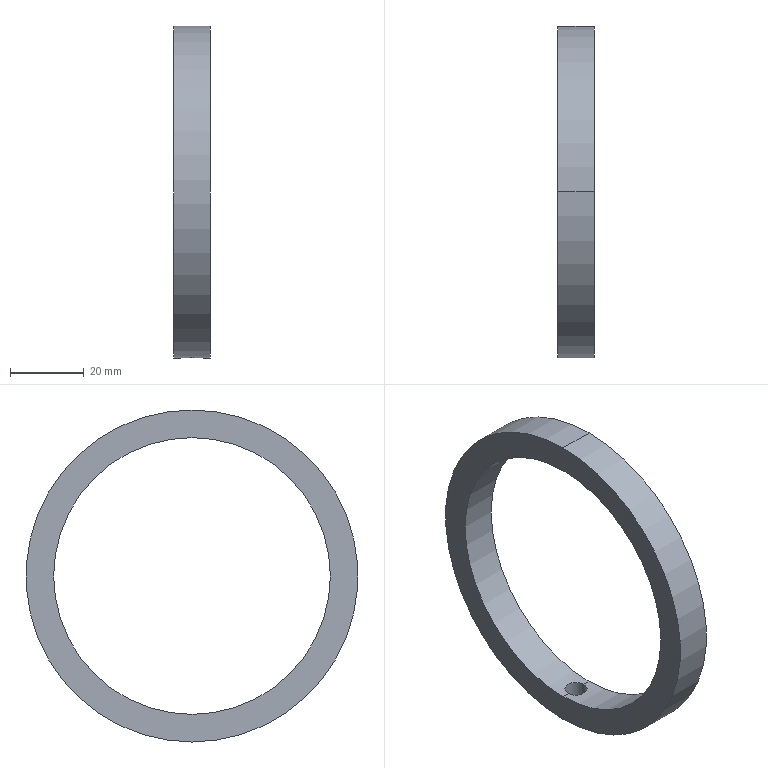Component | SolidWorks | 21Spacer-1 | 1 solid | 8 faces | box 10 x 90 x 90 mm | volume 19226 mm3 | cylinder 6 | plane 2 | commonest cylinder face diameters 6 x2 75 x2 90 x2
build123d program:
from build123d import *

# Parameters (mm, degrees)
SKETCH20_R          = 45
SKETCH20_R_2        = 37.5
BOSS_EXTRUDE7_DEPTH = 5
SKETCH21_R          = 3
CUT_EXTRUDE9_DEPTH  = 64.836


with BuildPart() as part:
    # Sketch20 → Boss-Extrude7 (new, symmetric)
    with BuildSketch(Plane(origin=(0, 0, 0), x_dir=(0, 0, -1), z_dir=(1, 0, 0))):
        Circle(SKETCH20_R)
        Circle(SKETCH20_R_2, mode=Mode.SUBTRACT)
    extrude(amount=BOSS_EXTRUDE7_DEPTH, both=True)

    # Sketch21 → Cut-Extrude9 (cut, through all)
    with BuildSketch(Plane.XY):
        Circle(SKETCH21_R)
    extrude(amount=-CUT_EXTRUDE9_DEPTH, mode=Mode.SUBTRACT)


solid = part.part

# Placed as in the assembly
solid = solid.moved(Location((-35.043, 1.776, 250), (0, 0, 0)))
STEP:
#1=COLOUR_RGB('',0.7922,0.8196,0.9333);
#2=FILL_AREA_STYLE_COLOUR('',#1);
#3=FILL_AREA_STYLE('',(#2));
#4=SURFACE_STYLE_FILL_AREA(#3);
#5=SURFACE_SIDE_STYLE('',(#4));
#6=SURFACE_STYLE_USAGE(.BOTH.,#5);
#7=PRESENTATION_STYLE_ASSIGNMENT((#6));
#8=CARTESIAN_POINT('',(-1.498,0.06992,8.071));
#9=VERTEX_POINT('',#8);
#10=CARTESIAN_POINT('',(-1.262,0.06992,8.071));
#11=VERTEX_POINT('',#10);
#12=CARTESIAN_POINT('',(-1.498,0.06992,8.071));
#13=CARTESIAN_POINT('',(-1.498,0.06221,8.071));
#14=CARTESIAN_POINT('',(-1.497,0.05455,8.071));
#15=CARTESIAN_POINT('',(-1.494,0.03932,8.071));
#16=CARTESIAN_POINT('',(-1.492,0.03186,8.071));
#17=CARTESIAN_POINT('',(-1.486,0.01765,8.072));
#18=CARTESIAN_POINT('',(-1.482,0.01079,8.072));
#19=CARTESIAN_POINT('',(-1.474,-0.00214,8.072));
#20=CARTESIAN_POINT('',(-1.469,-0.008088,8.073));
#21=CARTESIAN_POINT('',(-1.458,-0.01898,8.073));
#22=CARTESIAN_POINT('',(-1.452,-0.02397,8.073));
#23=CARTESIAN_POINT('',(-1.439,-0.03256,8.074));
#24=CARTESIAN_POINT('',(-1.432,-0.03619,8.074));
#25=CARTESIAN_POINT('',(-1.418,-0.04212,8.074));
#26=CARTESIAN_POINT('',(-1.41,-0.0444,8.075));
#27=CARTESIAN_POINT('',(-1.395,-0.04741,8.075));
#28=CARTESIAN_POINT('',(-1.388,-0.04818,8.075));
#29=CARTESIAN_POINT('',(-1.372,-0.04819,8.075));
#30=CARTESIAN_POINT('',(-1.364,-0.04743,8.075));
#31=CARTESIAN_POINT('',(-1.349,-0.04444,8.075));
#32=CARTESIAN_POINT('',(-1.342,-0.04218,8.074));
#33=CARTESIAN_POINT('',(-1.327,-0.03626,8.074));
#34=CARTESIAN_POINT('',(-1.321,-0.03264,8.074));
#35=CARTESIAN_POINT('',(-1.308,-0.02408,8.073));
#36=CARTESIAN_POINT('',(-1.302,-0.0191,8.073));
#37=CARTESIAN_POINT('',(-1.291,-0.008208,8.073));
#38=CARTESIAN_POINT('',(-1.286,-0.002269,8.072));
#39=CARTESIAN_POINT('',(-1.277,0.01062,8.072));
#40=CARTESIAN_POINT('',(-1.274,0.0175,8.072));
#41=CARTESIAN_POINT('',(-1.265,0.03881,8.071));
#42=CARTESIAN_POINT('',(-1.262,0.05431,8.071));
#43=CARTESIAN_POINT('',(-1.262,0.06992,8.071));
#44=B_SPLINE_CURVE_WITH_KNOTS('',3,(#12,#13,#14,#15,#16,#17,#18,#19,#20,#21,#22,#23,#24,#25,#26,#27,#28,#29,#30,#31,#32,#33,#34,#35,#36,#37,#38,#39,#40,#41,#42,#43),.UNSPECIFIED.,.F.,.F.,(4,2,2,2,2,2,2,2,2,2,2,2,2,2,2,4),(0.009382,0.009968,0.01055,0.01114,0.01173,0.01231,0.0129,0.01349,0.01407,0.01466,0.01524,0.01583,0.01642,0.017,0.01759,0.01876),.UNSPECIFIED.);
#45=EDGE_CURVE('',#9,#11,#44,.T.);
#46=ORIENTED_EDGE('',*,*,#45,.F.);
#47=CARTESIAN_POINT('',(-1.498,0.06992,8.366));
#48=VERTEX_POINT('',#47);
#49=CARTESIAN_POINT('',(-1.498,0.06992,8.071));
#50=DIRECTION('',(0.,0.,1.));
#51=VECTOR('',#50,39.37);
#52=LINE('',#49,#51);
#53=EDGE_CURVE('',#9,#48,#52,.T.);
#54=ORIENTED_EDGE('',*,*,#53,.T.);
#55=CARTESIAN_POINT('',(-1.262,0.06992,8.366));
#56=VERTEX_POINT('',#55);
#57=CARTESIAN_POINT('',(-1.498,0.06992,8.366));
#58=CARTESIAN_POINT('',(-1.498,0.06221,8.366));
#59=CARTESIAN_POINT('',(-1.497,0.05455,8.366));
#60=CARTESIAN_POINT('',(-1.494,0.03932,8.366));
#61=CARTESIAN_POINT('',(-1.492,0.03186,8.367));
#62=CARTESIAN_POINT('',(-1.486,0.01764,8.367));
#63=CARTESIAN_POINT('',(-1.482,0.01078,8.367));
#64=CARTESIAN_POINT('',(-1.474,-0.002141,8.368));
#65=CARTESIAN_POINT('',(-1.469,-0.008088,8.368));
#66=CARTESIAN_POINT('',(-1.458,-0.01898,8.369));
#67=CARTESIAN_POINT('',(-1.452,-0.02397,8.369));
#68=CARTESIAN_POINT('',(-1.439,-0.03255,8.37));
#69=CARTESIAN_POINT('',(-1.432,-0.03618,8.37));
#70=CARTESIAN_POINT('',(-1.418,-0.04212,8.37));
#71=CARTESIAN_POINT('',(-1.41,-0.0444,8.371));
#72=CARTESIAN_POINT('',(-1.395,-0.04741,8.371));
#73=CARTESIAN_POINT('',(-1.388,-0.04818,8.371));
#74=CARTESIAN_POINT('',(-1.372,-0.04819,8.371));
#75=CARTESIAN_POINT('',(-1.364,-0.04743,8.371));
#76=CARTESIAN_POINT('',(-1.349,-0.04444,8.371));
#77=CARTESIAN_POINT('',(-1.342,-0.04218,8.37));
#78=CARTESIAN_POINT('',(-1.327,-0.03626,8.37));
#79=CARTESIAN_POINT('',(-1.321,-0.03263,8.37));
#80=CARTESIAN_POINT('',(-1.308,-0.02408,8.369));
#81=CARTESIAN_POINT('',(-1.302,-0.0191,8.369));
#82=CARTESIAN_POINT('',(-1.291,-0.008209,8.368));
#83=CARTESIAN_POINT('',(-1.286,-0.002271,8.368));
#84=CARTESIAN_POINT('',(-1.277,0.01062,8.367));
#85=CARTESIAN_POINT('',(-1.274,0.0175,8.367));
#86=CARTESIAN_POINT('',(-1.265,0.0388,8.366));
#87=CARTESIAN_POINT('',(-1.262,0.05431,8.366));
#88=CARTESIAN_POINT('',(-1.262,0.06992,8.366));
#89=B_SPLINE_CURVE_WITH_KNOTS('',3,(#57,#58,#59,#60,#61,#62,#63,#64,#65,#66,#67,#68,#69,#70,#71,#72,#73,#74,#75,#76,#77,#78,#79,#80,#81,#82,#83,#84,#85,#86,#87,#88),.UNSPECIFIED.,.F.,.F.,(4,2,2,2,2,2,2,2,2,2,2,2,2,2,2,4),(0.009383,0.009969,0.01056,0.01114,0.01173,0.01231,0.0129,0.01349,0.01407,0.01466,0.01525,0.01583,0.01642,0.01701,0.01759,0.01876),.UNSPECIFIED.);
#90=EDGE_CURVE('',#48,#56,#89,.T.);
#91=ORIENTED_EDGE('',*,*,#90,.T.);
#92=CARTESIAN_POINT('',(-1.262,0.06992,8.071));
#93=DIRECTION('',(0.,0.,1.));
#94=VECTOR('',#93,39.37);
#95=LINE('',#92,#94);
#96=EDGE_CURVE('',#11,#56,#95,.T.);
#97=ORIENTED_EDGE('',*,*,#96,.F.);
#98=EDGE_LOOP('',(#46,#54,#91,#97));
#99=FACE_OUTER_BOUND('',#98,.T.);
#100=CARTESIAN_POINT('',(-1.38,0.06992,8.071));
#101=DIRECTION('',(0.,0.,1.));
#102=DIRECTION('',(1.,0.,0.));
#103=AXIS2_PLACEMENT_3D('',#100,#101,#102);
#104=CYLINDRICAL_SURFACE('',#103,0.1181);
#105=ADVANCED_FACE('',(#99),#104,.F.);
#106=CARTESIAN_POINT('',(-1.183,0.06992,11.319));
#107=VERTEX_POINT('',#106);
#108=CARTESIAN_POINT('',(-1.183,0.06992,8.366));
#109=VERTEX_POINT('',#108);
#110=CARTESIAN_POINT('',(-1.183,0.06992,9.843));
#111=DIRECTION('',(1.,0.,0.));
#112=DIRECTION('',(0.,0.,-1.));
#113=AXIS2_PLACEMENT_3D('',#110,#111,#112);
#114=CIRCLE('',#113,1.476);
#115=EDGE_CURVE('',#107,#109,#114,.T.);
#116=ORIENTED_EDGE('',*,*,#115,.T.);
#117=CARTESIAN_POINT('',(-1.183,0.06992,8.366));
#118=DIRECTION('',(-1.,0.,0.));
#119=VECTOR('',#118,39.37);
#120=LINE('',#117,#119);
#121=EDGE_CURVE('',#109,#56,#120,.T.);
#122=ORIENTED_EDGE('',*,*,#121,.T.);
#123=ORIENTED_EDGE('',*,*,#90,.F.);
#124=CARTESIAN_POINT('',(-1.576,0.06992,8.366));
#125=VERTEX_POINT('',#124);
#126=CARTESIAN_POINT('',(-1.183,0.06992,8.366));
#127=DIRECTION('',(-1.,0.,0.));
#128=VECTOR('',#127,39.37);
#129=LINE('',#126,#128);
#130=EDGE_CURVE('',#48,#125,#129,.T.);
#131=ORIENTED_EDGE('',*,*,#130,.T.);
#132=CARTESIAN_POINT('',(-1.576,0.06992,11.319));
#133=VERTEX_POINT('',#132);
#134=CARTESIAN_POINT('',(-1.576,0.06992,9.843));
#135=DIRECTION('',(1.,0.,0.));
#136=DIRECTION('',(0.,0.,-1.));
#137=AXIS2_PLACEMENT_3D('',#134,#135,#136);
#138=CIRCLE('',#137,1.476);
#139=EDGE_CURVE('',#133,#125,#138,.T.);
#140=ORIENTED_EDGE('',*,*,#139,.F.);
#141=CARTESIAN_POINT('',(-1.183,0.06992,11.319));
#142=DIRECTION('',(-1.,0.,0.));
#143=VECTOR('',#142,39.37);
#144=LINE('',#141,#143);
#145=EDGE_CURVE('',#107,#133,#144,.T.);
#146=ORIENTED_EDGE('',*,*,#145,.F.);
#147=EDGE_LOOP('',(#116,#122,#123,#131,#140,#146));
#148=FACE_OUTER_BOUND('',#147,.T.);
#149=CARTESIAN_POINT('',(-1.183,0.06992,9.843));
#150=DIRECTION('',(-1.,0.,0.));
#151=DIRECTION('',(0.,0.,1.));
#152=AXIS2_PLACEMENT_3D('',#149,#150,#151);
#153=CYLINDRICAL_SURFACE('',#152,1.476);
#154=ADVANCED_FACE('',(#148),#153,.F.);
#155=CARTESIAN_POINT('',(-1.183,0.06992,8.071));
#156=VERTEX_POINT('',#155);
#157=CARTESIAN_POINT('',(-1.183,0.06992,11.614));
#158=VERTEX_POINT('',#157);
#159=CARTESIAN_POINT('',(-1.183,0.06992,9.843));
#160=DIRECTION('',(1.,0.,0.));
#161=DIRECTION('',(0.,0.,-1.));
#162=AXIS2_PLACEMENT_3D('',#159,#160,#161);
#163=CIRCLE('',#162,1.772);
#164=EDGE_CURVE('',#156,#158,#163,.T.);
#165=ORIENTED_EDGE('',*,*,#164,.F.);
#166=CARTESIAN_POINT('',(-1.183,0.06992,8.071));
#167=DIRECTION('',(-1.,0.,0.));
#168=VECTOR('',#167,39.37);
#169=LINE('',#166,#168);
#170=EDGE_CURVE('',#156,#11,#169,.T.);
#171=ORIENTED_EDGE('',*,*,#170,.T.);
#172=CARTESIAN_POINT('',(-1.262,0.06992,8.071));
#173=CARTESIAN_POINT('',(-1.262,0.07773,8.071));
#174=CARTESIAN_POINT('',(-1.262,0.0854,8.071));
#175=CARTESIAN_POINT('',(-1.265,0.1005,8.071));
#176=CARTESIAN_POINT('',(-1.268,0.108,8.071));
#177=CARTESIAN_POINT('',(-1.273,0.1223,8.072));
#178=CARTESIAN_POINT('',(-1.277,0.1291,8.072));
#179=CARTESIAN_POINT('',(-1.286,0.1419,8.072));
#180=CARTESIAN_POINT('',(-1.291,0.148,8.073));
#181=CARTESIAN_POINT('',(-1.302,0.1589,8.073));
#182=CARTESIAN_POINT('',(-1.308,0.1638,8.073));
#183=CARTESIAN_POINT('',(-1.32,0.1724,8.074));
#184=CARTESIAN_POINT('',(-1.327,0.1761,8.074));
#185=CARTESIAN_POINT('',(-1.342,0.182,8.074));
#186=CARTESIAN_POINT('',(-1.349,0.1842,8.075));
#187=CARTESIAN_POINT('',(-1.364,0.1873,8.075));
#188=CARTESIAN_POINT('',(-1.372,0.188,8.075));
#189=CARTESIAN_POINT('',(-1.387,0.188,8.075));
#190=CARTESIAN_POINT('',(-1.395,0.1873,8.075));
#191=CARTESIAN_POINT('',(-1.41,0.1843,8.075));
#192=CARTESIAN_POINT('',(-1.418,0.182,8.074));
#193=CARTESIAN_POINT('',(-1.432,0.1761,8.074));
#194=CARTESIAN_POINT('',(-1.439,0.1724,8.074));
#195=CARTESIAN_POINT('',(-1.452,0.1639,8.073));
#196=CARTESIAN_POINT('',(-1.458,0.159,8.073));
#197=CARTESIAN_POINT('',(-1.469,0.1479,8.073));
#198=CARTESIAN_POINT('',(-1.474,0.142,8.072));
#199=CARTESIAN_POINT('',(-1.482,0.1292,8.072));
#200=CARTESIAN_POINT('',(-1.486,0.1223,8.072));
#201=CARTESIAN_POINT('',(-1.492,0.108,8.071));
#202=CARTESIAN_POINT('',(-1.494,0.1006,8.071));
#203=CARTESIAN_POINT('',(-1.497,0.08546,8.071));
#204=CARTESIAN_POINT('',(-1.498,0.07763,8.071));
#205=CARTESIAN_POINT('',(-1.498,0.06992,8.071));
#206=B_SPLINE_CURVE_WITH_KNOTS('',3,(#172,#173,#174,#175,#176,#177,#178,#179,#180,#181,#182,#183,#184,#185,#186,#187,#188,#189,#190,#191,#192,#193,#194,#195,#196,#197,#198,#199,#200,#201,#202,#203,#204,#205),.UNSPECIFIED.,.F.,.F.,(4,2,2,2,2,2,2,2,2,2,2,2,2,2,2,2,4),(0.,0.0005864,0.001173,0.001759,0.002345,0.002932,0.003518,0.004105,0.004691,0.005277,0.005864,0.00645,0.007036,0.007623,0.008209,0.008796,0.009382),.UNSPECIFIED.);
#207=EDGE_CURVE('',#11,#9,#206,.T.);
#208=ORIENTED_EDGE('',*,*,#207,.T.);
#209=CARTESIAN_POINT('',(-1.576,0.06992,8.071));
#210=VERTEX_POINT('',#209);
#211=CARTESIAN_POINT('',(-1.183,0.06992,8.071));
#212=DIRECTION('',(-1.,0.,0.));
#213=VECTOR('',#212,39.37);
#214=LINE('',#211,#213);
#215=EDGE_CURVE('',#9,#210,#214,.T.);
#216=ORIENTED_EDGE('',*,*,#215,.T.);
#217=CARTESIAN_POINT('',(-1.576,0.06992,11.614));
#218=VERTEX_POINT('',#217);
#219=CARTESIAN_POINT('',(-1.576,0.06992,9.843));
#220=DIRECTION('',(1.,0.,0.));
#221=DIRECTION('',(0.,0.,-1.));
#222=AXIS2_PLACEMENT_3D('',#219,#220,#221);
#223=CIRCLE('',#222,1.772);
#224=EDGE_CURVE('',#210,#218,#223,.T.);
#225=ORIENTED_EDGE('',*,*,#224,.T.);
#226=CARTESIAN_POINT('',(-1.183,0.06992,11.614));
#227=DIRECTION('',(-1.,0.,0.));
#228=VECTOR('',#227,39.37);
#229=LINE('',#226,#228);
#230=EDGE_CURVE('',#158,#218,#229,.T.);
#231=ORIENTED_EDGE('',*,*,#230,.F.);
#232=EDGE_LOOP('',(#165,#171,#208,#216,#225,#231));
#233=FACE_OUTER_BOUND('',#232,.T.);
#234=CARTESIAN_POINT('',(-1.183,0.06992,9.843));
#235=DIRECTION('',(-1.,0.,0.));
#236=DIRECTION('',(0.,0.,1.));
#237=AXIS2_PLACEMENT_3D('',#234,#235,#236);
#238=CYLINDRICAL_SURFACE('',#237,1.772);
#239=ADVANCED_FACE('',(#233),#238,.T.);
#240=CARTESIAN_POINT('',(-1.183,0.06992,9.843));
#241=DIRECTION('',(1.,0.,0.));
#242=DIRECTION('',(0.,0.,-1.));
#243=AXIS2_PLACEMENT_3D('',#240,#241,#242);
#244=CIRCLE('',#243,1.772);
#245=EDGE_CURVE('',#158,#156,#244,.T.);
#246=ORIENTED_EDGE('',*,*,#245,.T.);
#247=ORIENTED_EDGE('',*,*,#164,.T.);
#248=EDGE_LOOP('',(#246,#247));
#249=FACE_OUTER_BOUND('',#248,.T.);
#250=ORIENTED_EDGE('',*,*,#115,.F.);
#251=CARTESIAN_POINT('',(-1.183,0.06992,9.843));
#252=DIRECTION('',(1.,0.,0.));
#253=DIRECTION('',(0.,0.,-1.));
#254=AXIS2_PLACEMENT_3D('',#251,#252,#253);
#255=CIRCLE('',#254,1.476);
#256=EDGE_CURVE('',#109,#107,#255,.T.);
#257=ORIENTED_EDGE('',*,*,#256,.F.);
#258=EDGE_LOOP('',(#250,#257));
#259=FACE_BOUND('',#258,.T.);
#260=CARTESIAN_POINT('',(-1.183,0.06992,9.843));
#261=DIRECTION('',(1.,0.,0.));
#262=DIRECTION('',(0.,0.,-1.));
#263=AXIS2_PLACEMENT_3D('',#260,#261,#262);
#264=PLANE('',#263);
#265=ADVANCED_FACE('',(#249,#259),#264,.T.);
#266=CARTESIAN_POINT('',(-1.576,0.06992,9.843));
#267=DIRECTION('',(1.,0.,0.));
#268=DIRECTION('',(0.,0.,-1.));
#269=AXIS2_PLACEMENT_3D('',#266,#267,#268);
#270=CIRCLE('',#269,1.772);
#271=EDGE_CURVE('',#218,#210,#270,.T.);
#272=ORIENTED_EDGE('',*,*,#271,.F.);
#273=ORIENTED_EDGE('',*,*,#224,.F.);
#274=EDGE_LOOP('',(#272,#273));
#275=FACE_OUTER_BOUND('',#274,.T.);
#276=ORIENTED_EDGE('',*,*,#139,.T.);
#277=CARTESIAN_POINT('',(-1.576,0.06992,9.843));
#278=DIRECTION('',(1.,0.,0.));
#279=DIRECTION('',(0.,0.,-1.));
#280=AXIS2_PLACEMENT_3D('',#277,#278,#279);
#281=CIRCLE('',#280,1.476);
#282=EDGE_CURVE('',#125,#133,#281,.T.);
#283=ORIENTED_EDGE('',*,*,#282,.T.);
#284=EDGE_LOOP('',(#276,#283));
#285=FACE_BOUND('',#284,.T.);
#286=CARTESIAN_POINT('',(-1.576,0.06992,9.843));
#287=DIRECTION('',(1.,0.,0.));
#288=DIRECTION('',(0.,0.,-1.));
#289=AXIS2_PLACEMENT_3D('',#286,#287,#288);
#290=PLANE('',#289);
#291=ADVANCED_FACE('',(#275,#285),#290,.F.);
#292=ORIENTED_EDGE('',*,*,#170,.F.);
#293=ORIENTED_EDGE('',*,*,#245,.F.);
#294=ORIENTED_EDGE('',*,*,#230,.T.);
#295=ORIENTED_EDGE('',*,*,#271,.T.);
#296=ORIENTED_EDGE('',*,*,#215,.F.);
#297=ORIENTED_EDGE('',*,*,#45,.T.);
#298=EDGE_LOOP('',(#292,#293,#294,#295,#296,#297));
#299=FACE_OUTER_BOUND('',#298,.T.);
#300=CARTESIAN_POINT('',(-1.183,0.06992,9.843));
#301=DIRECTION('',(-1.,0.,0.));
#302=DIRECTION('',(0.,0.,1.));
#303=AXIS2_PLACEMENT_3D('',#300,#301,#302);
#304=CYLINDRICAL_SURFACE('',#303,1.772);
#305=ADVANCED_FACE('',(#299),#304,.T.);
#306=ORIENTED_EDGE('',*,*,#121,.F.);
#307=ORIENTED_EDGE('',*,*,#256,.T.);
#308=ORIENTED_EDGE('',*,*,#145,.T.);
#309=ORIENTED_EDGE('',*,*,#282,.F.);
#310=ORIENTED_EDGE('',*,*,#130,.F.);
#311=CARTESIAN_POINT('',(-1.262,0.06992,8.366));
#312=CARTESIAN_POINT('',(-1.262,0.07773,8.366));
#313=CARTESIAN_POINT('',(-1.262,0.08541,8.366));
#314=CARTESIAN_POINT('',(-1.265,0.1005,8.366));
#315=CARTESIAN_POINT('',(-1.268,0.108,8.367));
#316=CARTESIAN_POINT('',(-1.273,0.1223,8.367));
#317=CARTESIAN_POINT('',(-1.277,0.1291,8.367));
#318=CARTESIAN_POINT('',(-1.286,0.1419,8.368));
#319=CARTESIAN_POINT('',(-1.291,0.148,8.368));
#320=CARTESIAN_POINT('',(-1.302,0.1589,8.369));
#321=CARTESIAN_POINT('',(-1.308,0.1638,8.369));
#322=CARTESIAN_POINT('',(-1.32,0.1724,8.37));
#323=CARTESIAN_POINT('',(-1.327,0.1761,8.37));
#324=CARTESIAN_POINT('',(-1.342,0.182,8.37));
#325=CARTESIAN_POINT('',(-1.349,0.1842,8.371));
#326=CARTESIAN_POINT('',(-1.364,0.1873,8.371));
#327=CARTESIAN_POINT('',(-1.372,0.188,8.371));
#328=CARTESIAN_POINT('',(-1.387,0.188,8.371));
#329=CARTESIAN_POINT('',(-1.395,0.1873,8.371));
#330=CARTESIAN_POINT('',(-1.41,0.1842,8.371));
#331=CARTESIAN_POINT('',(-1.418,0.182,8.37));
#332=CARTESIAN_POINT('',(-1.432,0.1761,8.37));
#333=CARTESIAN_POINT('',(-1.439,0.1724,8.37));
#334=CARTESIAN_POINT('',(-1.452,0.1638,8.369));
#335=CARTESIAN_POINT('',(-1.458,0.159,8.369));
#336=CARTESIAN_POINT('',(-1.469,0.1479,8.368));
#337=CARTESIAN_POINT('',(-1.474,0.142,8.368));
#338=CARTESIAN_POINT('',(-1.482,0.1292,8.367));
#339=CARTESIAN_POINT('',(-1.486,0.1223,8.367));
#340=CARTESIAN_POINT('',(-1.492,0.108,8.367));
#341=CARTESIAN_POINT('',(-1.494,0.1006,8.366));
#342=CARTESIAN_POINT('',(-1.497,0.08546,8.366));
#343=CARTESIAN_POINT('',(-1.498,0.07763,8.366));
#344=CARTESIAN_POINT('',(-1.498,0.06992,8.366));
#345=B_SPLINE_CURVE_WITH_KNOTS('',3,(#311,#312,#313,#314,#315,#316,#317,#318,#319,#320,#321,#322,#323,#324,#325,#326,#327,#328,#329,#330,#331,#332,#333,#334,#335,#336,#337,#338,#339,#340,#341,#342,#343,#344),.UNSPECIFIED.,.F.,.F.,(4,2,2,2,2,2,2,2,2,2,2,2,2,2,2,2,4),(0.,0.0005864,0.001173,0.001759,0.002346,0.002932,0.003519,0.004105,0.004692,0.005278,0.005864,0.006451,0.007037,0.007624,0.00821,0.008797,0.009383),.UNSPECIFIED.);
#346=EDGE_CURVE('',#56,#48,#345,.T.);
#347=ORIENTED_EDGE('',*,*,#346,.F.);
#348=EDGE_LOOP('',(#306,#307,#308,#309,#310,#347));
#349=FACE_OUTER_BOUND('',#348,.T.);
#350=CARTESIAN_POINT('',(-1.183,0.06992,9.843));
#351=DIRECTION('',(-1.,0.,0.));
#352=DIRECTION('',(0.,0.,1.));
#353=AXIS2_PLACEMENT_3D('',#350,#351,#352);
#354=CYLINDRICAL_SURFACE('',#353,1.476);
#355=ADVANCED_FACE('',(#349),#354,.F.);
#356=ORIENTED_EDGE('',*,*,#53,.F.);
#357=ORIENTED_EDGE('',*,*,#207,.F.);
#358=ORIENTED_EDGE('',*,*,#96,.T.);
#359=ORIENTED_EDGE('',*,*,#346,.T.);
#360=EDGE_LOOP('',(#356,#357,#358,#359));
#361=FACE_OUTER_BOUND('',#360,.T.);
#362=CARTESIAN_POINT('',(-1.38,0.06992,8.071));
#363=DIRECTION('',(0.,0.,1.));
#364=DIRECTION('',(1.,0.,0.));
#365=AXIS2_PLACEMENT_3D('',#362,#363,#364);
#366=CYLINDRICAL_SURFACE('',#365,0.1181);
#367=ADVANCED_FACE('',(#361),#366,.F.);
#368=CLOSED_SHELL('',(#105,#154,#239,#265,#291,#305,#355,#367));
#369=MANIFOLD_SOLID_BREP('',#368);
#370=STYLED_ITEM('',(#7),#369);
#371=(LENGTH_UNIT()NAMED_UNIT(*)SI_UNIT($,.METRE.));
#372=LENGTH_MEASURE_WITH_UNIT(LENGTH_MEASURE(0.0254),#371);
#373=DIMENSIONAL_EXPONENTS(1.,0.,0.,0.,0.,0.,0.);
#374=(CONVERSION_BASED_UNIT('',#372)LENGTH_UNIT()NAMED_UNIT(#373));
#375=UNCERTAINTY_MEASURE_WITH_UNIT(LENGTH_MEASURE(0.00001),#374,'','');
#376=(NAMED_UNIT(*)PLANE_ANGLE_UNIT()SI_UNIT($,.RADIAN.));
#377=(NAMED_UNIT(*)SI_UNIT($,.STERADIAN.)SOLID_ANGLE_UNIT());
#378=(GEOMETRIC_REPRESENTATION_CONTEXT(3)GLOBAL_UNCERTAINTY_ASSIGNED_CONTEXT((#375))GLOBAL_UNIT_ASSIGNED_CONTEXT((#374,#376,#377))REPRESENTATION_CONTEXT('',''));
#379=MECHANICAL_DESIGN_GEOMETRIC_PRESENTATION_REPRESENTATION('',(#370),#378);
#380=CARTESIAN_POINT('',(0.,0.,0.));
#381=DIRECTION('',(0.,0.,1.));
#382=DIRECTION('',(1.,0.,0.));
#383=AXIS2_PLACEMENT_3D('',#380,#381,#382);
#384=(LENGTH_UNIT()NAMED_UNIT(*)SI_UNIT($,.METRE.));
#385=LENGTH_MEASURE_WITH_UNIT(LENGTH_MEASURE(0.0254),#384);
#386=DIMENSIONAL_EXPONENTS(1.,0.,0.,0.,0.,0.,0.);
#387=(CONVERSION_BASED_UNIT('',#385)LENGTH_UNIT()NAMED_UNIT(#386));
#388=UNCERTAINTY_MEASURE_WITH_UNIT(LENGTH_MEASURE(0.00001),#387,'','');
#389=(NAMED_UNIT(*)PLANE_ANGLE_UNIT()SI_UNIT($,.RADIAN.));
#390=(NAMED_UNIT(*)SI_UNIT($,.STERADIAN.)SOLID_ANGLE_UNIT());
#391=(GEOMETRIC_REPRESENTATION_CONTEXT(3)GLOBAL_UNCERTAINTY_ASSIGNED_CONTEXT((#388))GLOBAL_UNIT_ASSIGNED_CONTEXT((#387,#389,#390))REPRESENTATION_CONTEXT('',''));
#392=ADVANCED_BREP_SHAPE_REPRESENTATION('',(#369,#383),#391);
#393=PRESENTATION_LAYER_ASSIGNMENT('','',(#370));